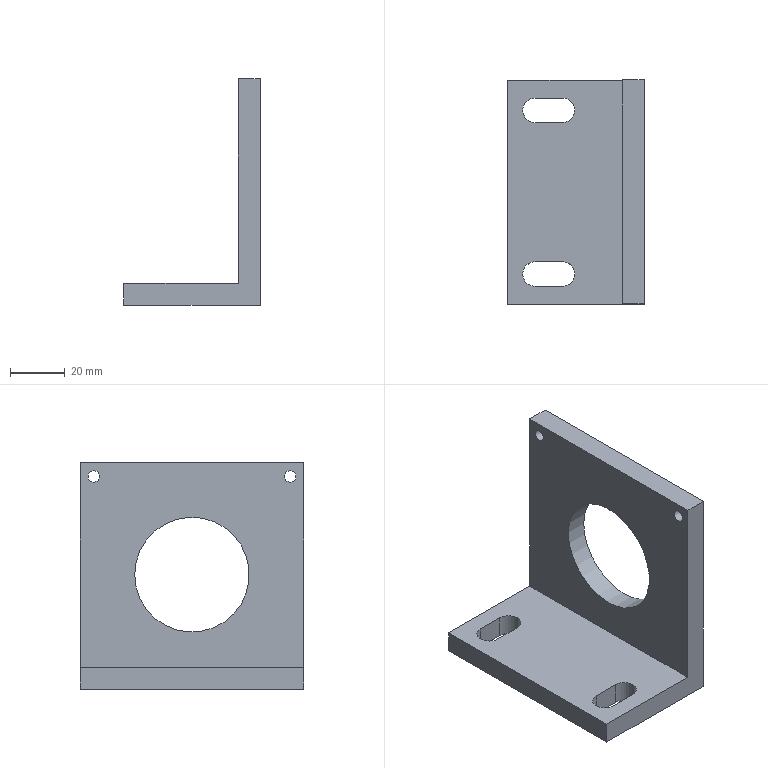Component | NX | MOTOR_BRACKET_2 | 1 solid | 23 faces | volume 68015 mm3 | plane 14 | cylinder 9 | commonest cylinder face diameters 4.2 x4 9 x4 42 x1